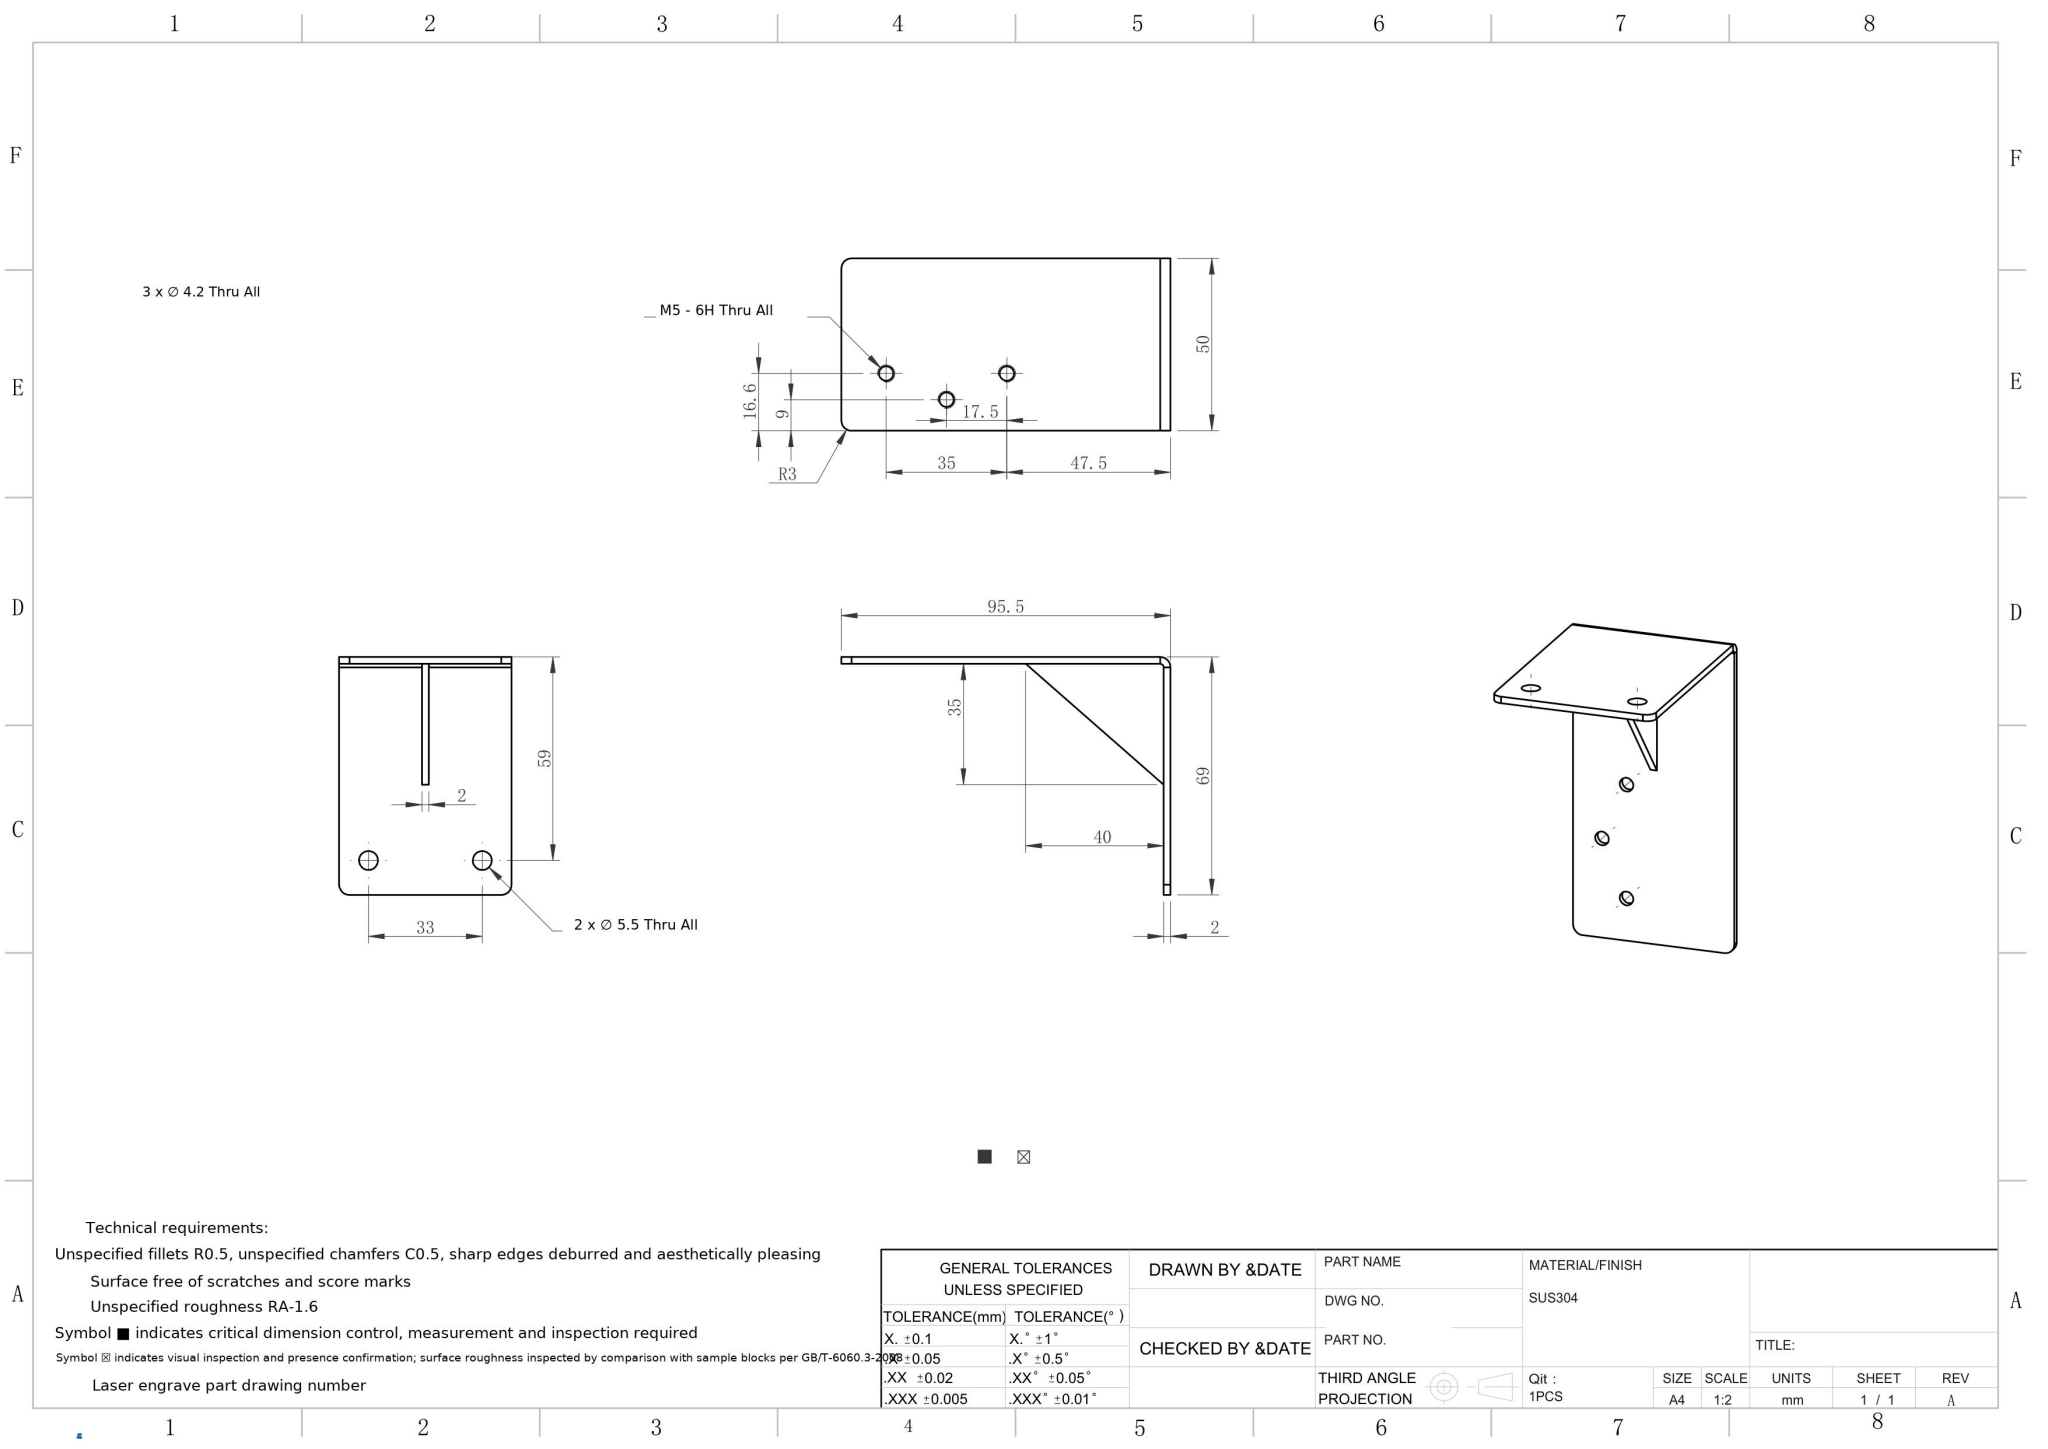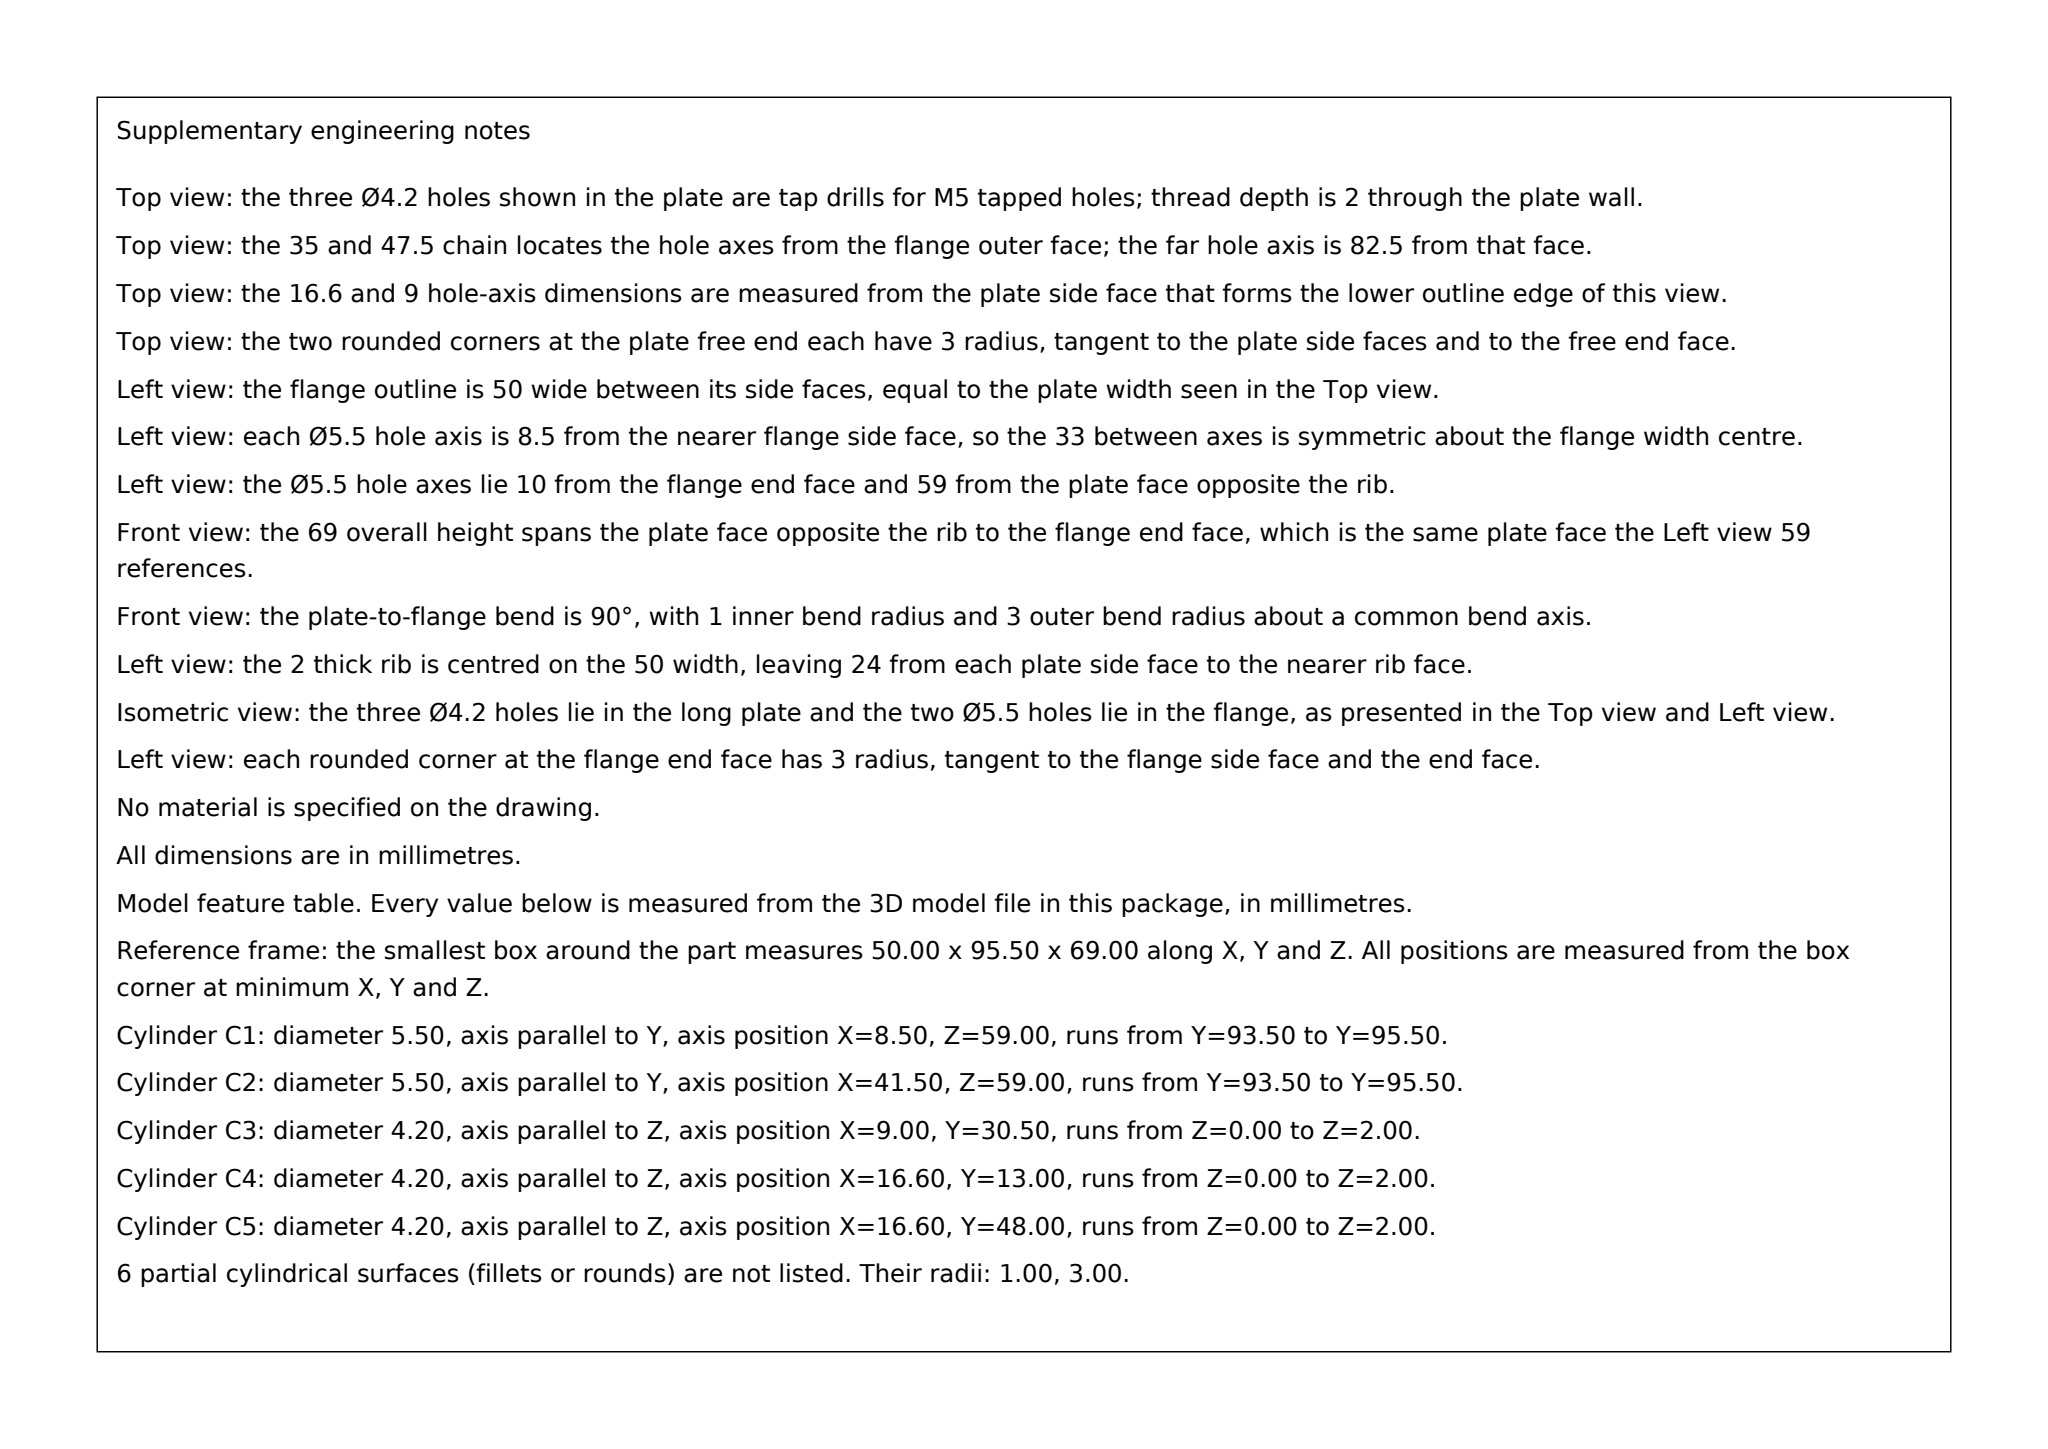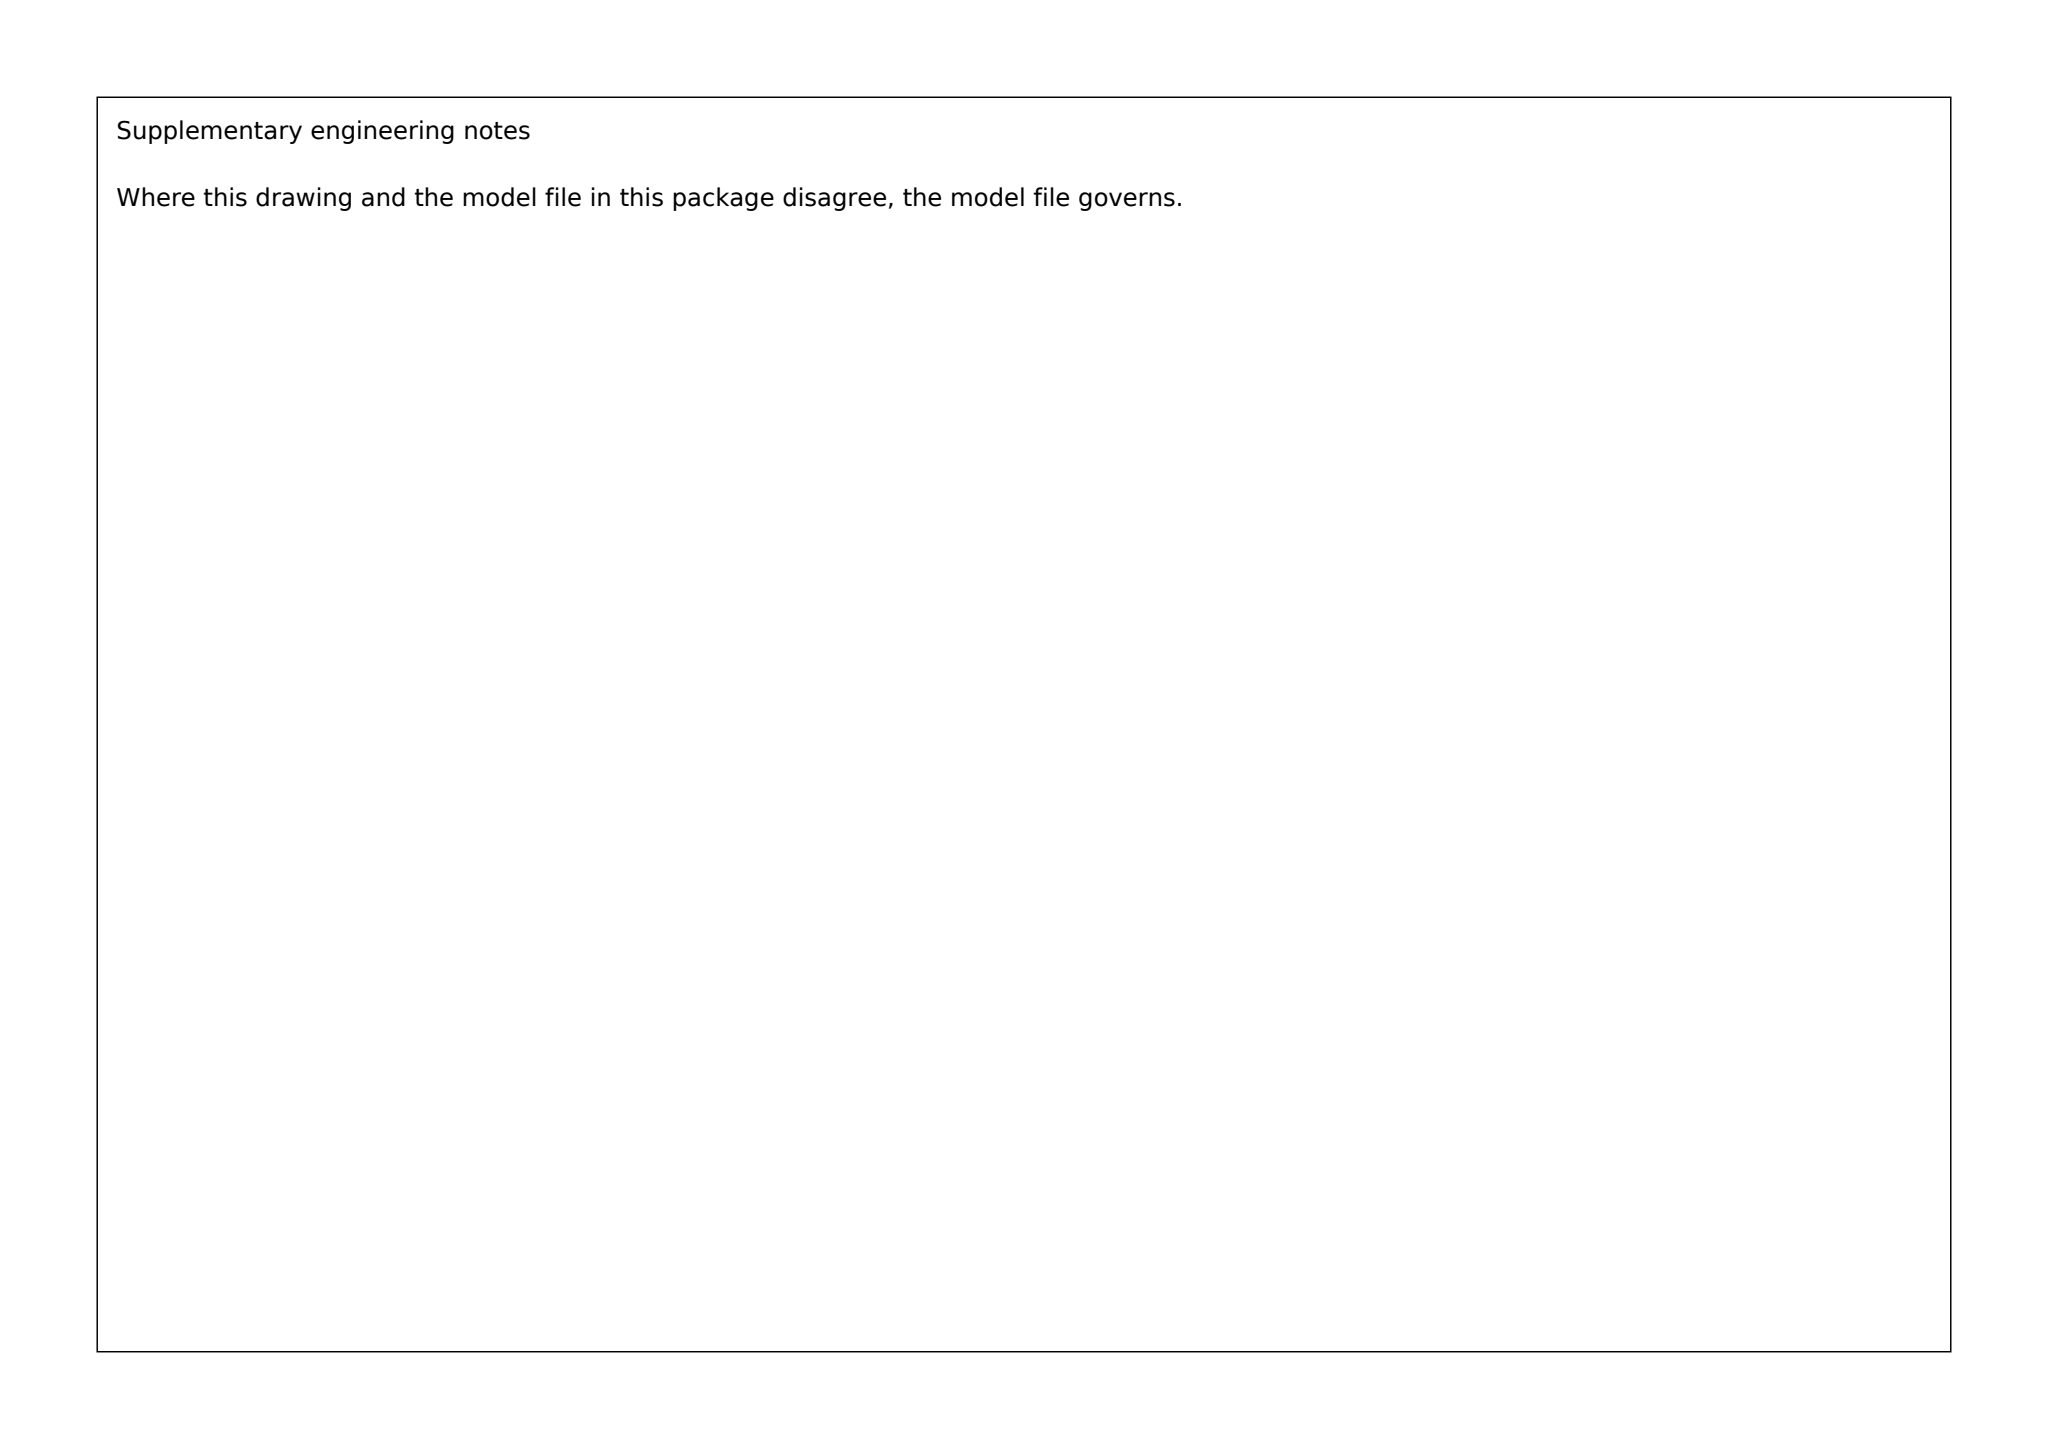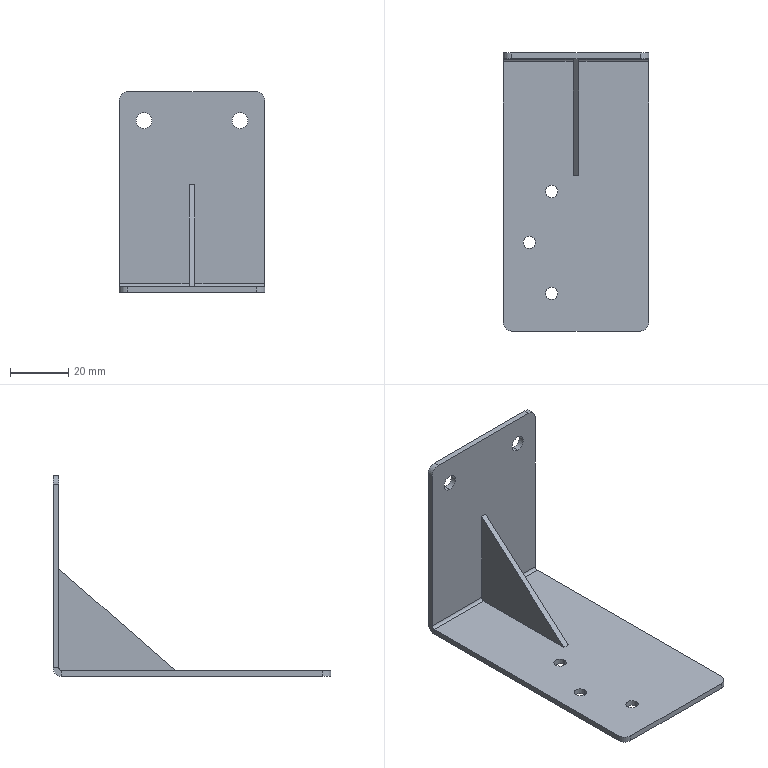Part | SolidWorks | mm | 1 solid | 32 faces | box 50 x 95.5 x 69 mm | volume 17370 mm3 | cylinder 17 | plane 15 | commonest cylinder face diameters 4.2 x6 6 x5 5.5 x4 2 x2
Drawing notes:
RIB 2 THK SYM ABT CL OF 50 WIDTH (24 & 26 FROM SIDE FACE) | from the solid: axis_planes x=24.0 and x=26.0 bound 2 thk rib; bbox x=50 -> rib centred, 24 from each side
2X Ø5.5 THRU: 8.5 FROM EA SIDE EDGE, SYM ABT CL (33 APART) | from the solid: cylinders Ø5.5 axis y at x=8.5 and x=41.5; bbox x=50 -> 8.5 edge dist each side
2X R3 AT FREE-END CNRS OF HORIZ PLATE | from the solid: Ø6 (R3) axis z cyls at (x=3,y=3) and (x=47,y=3), len 2 = horiz plate free end y=0